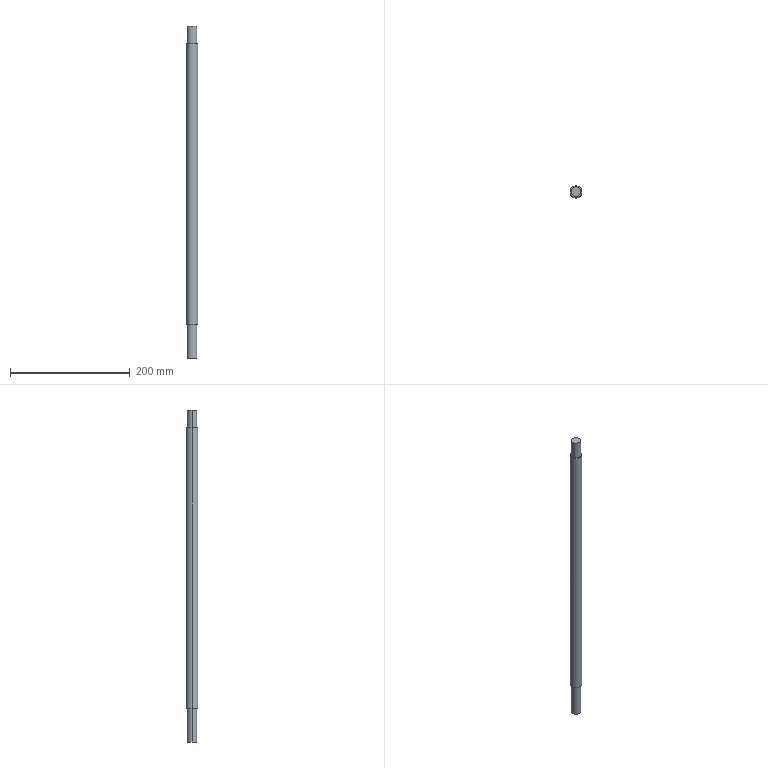Component | SolidWorks | LeadScrew-1 | 1 solid | 10 faces | box 20 x 20 x 555.57 mm | volume 164746 mm3 | cylinder 6 | plane 4 | commonest cylinder face diameters 16 x4 20 x2
build123d program:
from build123d import *

# Parameters (mm, degrees)
SKETCH1_R           = 10
BOSS_EXTRUDE1_DEPTH = 529
SKETCH2_R           = 10
SKETCH2_R_2         = 8
CUT_EXTRUDE1_DEPTH  = 30
CUT_EXTRUDE2_START  = -30
SKETCH3_R           = 10
SKETCH3_R_2         = 8
CUT_EXTRUDE2_DEPTH  = 30
MOVE_FACE1_BY       = 26.565


with BuildPart() as part:
    # Sketch1 → Boss-Extrude1 (new body)
    with BuildSketch(Plane.XY):
        with Locations((0, -208.707)):
            Circle(SKETCH1_R)
    extrude(amount=BOSS_EXTRUDE1_DEPTH)

    # Sketch2 → Cut-Extrude1 (cut)
    with BuildSketch(Plane(origin=(0, 0, 0), x_dir=(-1, 0, 0), z_dir=(0, 0, -1))):
        with Locations((0, -208.707)):
            Circle(SKETCH2_R)
        with Locations((0, -208.707)):
            Circle(SKETCH2_R_2, mode=Mode.SUBTRACT)
    extrude(amount=-CUT_EXTRUDE1_DEPTH, mode=Mode.SUBTRACT)

    # Sketch3 → Cut-Extrude2 (cut)
    with BuildSketch(Plane.XY.offset(529).offset(CUT_EXTRUDE2_START)):
        with Locations(Location((0, -208.707, 0), (0, 0, 180))):
            Circle(SKETCH3_R)
        with Locations(Location((0, -208.707, 0), (0, 0, 180))):
            Circle(SKETCH3_R_2, mode=Mode.SUBTRACT)
    extrude(amount=CUT_EXTRUDE2_DEPTH, mode=Mode.SUBTRACT)

    # Move Face1: a face moved outward by 26.565
    extrude(part.faces().sort_by_distance((0, -208.707, 529))[0], amount=MOVE_FACE1_BY, dir=(0, 0, 1))


solid = part.part

# Placed as in the assembly
solid = solid.moved(Location((0, -417.415, -102), (180, 0, 0)))
STEP:
#1=COLOUR_RGB('',0.7922,0.8196,0.9333);
#2=FILL_AREA_STYLE_COLOUR('',#1);
#3=FILL_AREA_STYLE('',(#2));
#4=SURFACE_STYLE_FILL_AREA(#3);
#5=SURFACE_SIDE_STYLE('',(#4));
#6=SURFACE_STYLE_USAGE(.BOTH.,#5);
#7=PRESENTATION_STYLE_ASSIGNMENT((#6));
#8=CARTESIAN_POINT('',(-0.315,-8.217,-23.661));
#9=VERTEX_POINT('',#8);
#10=CARTESIAN_POINT('',(0.315,-8.217,-23.661));
#11=VERTEX_POINT('',#10);
#12=CARTESIAN_POINT('',(0.,-8.217,-23.661));
#13=DIRECTION('',(0.,0.,-1.));
#14=DIRECTION('',(-1.,0.,0.));
#15=AXIS2_PLACEMENT_3D('',#12,#13,#14);
#16=CIRCLE('',#15,0.315);
#17=EDGE_CURVE('',#9,#11,#16,.T.);
#18=ORIENTED_EDGE('',*,*,#17,.T.);
#19=CARTESIAN_POINT('',(0.315,-8.217,-25.888));
#20=VERTEX_POINT('',#19);
#21=CARTESIAN_POINT('',(0.315,-8.217,-23.661));
#22=DIRECTION('',(0.,0.,-1.));
#23=VECTOR('',#22,39.37);
#24=LINE('',#21,#23);
#25=EDGE_CURVE('',#11,#20,#24,.T.);
#26=ORIENTED_EDGE('',*,*,#25,.T.);
#27=CARTESIAN_POINT('',(-0.315,-8.217,-25.888));
#28=VERTEX_POINT('',#27);
#29=CARTESIAN_POINT('',(0.,-8.217,-25.888));
#30=DIRECTION('',(0.,0.,-1.));
#31=DIRECTION('',(-1.,0.,0.));
#32=AXIS2_PLACEMENT_3D('',#29,#30,#31);
#33=CIRCLE('',#32,0.315);
#34=EDGE_CURVE('',#28,#20,#33,.T.);
#35=ORIENTED_EDGE('',*,*,#34,.F.);
#36=CARTESIAN_POINT('',(-0.315,-8.217,-23.661));
#37=DIRECTION('',(0.,0.,-1.));
#38=VECTOR('',#37,39.37);
#39=LINE('',#36,#38);
#40=EDGE_CURVE('',#9,#28,#39,.T.);
#41=ORIENTED_EDGE('',*,*,#40,.F.);
#42=EDGE_LOOP('',(#18,#26,#35,#41));
#43=FACE_OUTER_BOUND('',#42,.T.);
#44=CARTESIAN_POINT('',(0.,-8.217,-23.661));
#45=DIRECTION('',(0.,0.,-1.));
#46=DIRECTION('',(-1.,0.,0.));
#47=AXIS2_PLACEMENT_3D('',#44,#45,#46);
#48=CYLINDRICAL_SURFACE('',#47,0.315);
#49=ADVANCED_FACE('',(#43),#48,.T.);
#50=CARTESIAN_POINT('',(0.315,-8.217,-5.197));
#51=VERTEX_POINT('',#50);
#52=CARTESIAN_POINT('',(-0.315,-8.217,-5.197));
#53=VERTEX_POINT('',#52);
#54=CARTESIAN_POINT('',(0.,-8.217,-5.197));
#55=DIRECTION('',(0.,0.,1.));
#56=DIRECTION('',(1.,0.,0.));
#57=AXIS2_PLACEMENT_3D('',#54,#55,#56);
#58=CIRCLE('',#57,0.315);
#59=EDGE_CURVE('',#51,#53,#58,.T.);
#60=ORIENTED_EDGE('',*,*,#59,.T.);
#61=CARTESIAN_POINT('',(-0.315,-8.217,-4.016));
#62=VERTEX_POINT('',#61);
#63=CARTESIAN_POINT('',(-0.315,-8.217,-5.197));
#64=DIRECTION('',(0.,0.,1.));
#65=VECTOR('',#64,39.37);
#66=LINE('',#63,#65);
#67=EDGE_CURVE('',#53,#62,#66,.T.);
#68=ORIENTED_EDGE('',*,*,#67,.T.);
#69=CARTESIAN_POINT('',(0.315,-8.217,-4.016));
#70=VERTEX_POINT('',#69);
#71=CARTESIAN_POINT('',(0.,-8.217,-4.016));
#72=DIRECTION('',(0.,0.,1.));
#73=DIRECTION('',(1.,0.,0.));
#74=AXIS2_PLACEMENT_3D('',#71,#72,#73);
#75=CIRCLE('',#74,0.315);
#76=EDGE_CURVE('',#70,#62,#75,.T.);
#77=ORIENTED_EDGE('',*,*,#76,.F.);
#78=CARTESIAN_POINT('',(0.315,-8.217,-5.197));
#79=DIRECTION('',(0.,0.,1.));
#80=VECTOR('',#79,39.37);
#81=LINE('',#78,#80);
#82=EDGE_CURVE('',#51,#70,#81,.T.);
#83=ORIENTED_EDGE('',*,*,#82,.F.);
#84=EDGE_LOOP('',(#60,#68,#77,#83));
#85=FACE_OUTER_BOUND('',#84,.T.);
#86=CARTESIAN_POINT('',(0.,-8.217,-5.197));
#87=DIRECTION('',(0.,0.,1.));
#88=DIRECTION('',(1.,0.,0.));
#89=AXIS2_PLACEMENT_3D('',#86,#87,#88);
#90=CYLINDRICAL_SURFACE('',#89,0.315);
#91=ADVANCED_FACE('',(#85),#90,.T.);
#92=CARTESIAN_POINT('',(-0.3937,-8.217,-23.661));
#93=VERTEX_POINT('',#92);
#94=CARTESIAN_POINT('',(0.3937,-8.217,-23.661));
#95=VERTEX_POINT('',#94);
#96=CARTESIAN_POINT('',(0.,-8.217,-23.661));
#97=DIRECTION('',(0.,0.,-1.));
#98=DIRECTION('',(-1.,0.,0.));
#99=AXIS2_PLACEMENT_3D('',#96,#97,#98);
#100=CIRCLE('',#99,0.3937);
#101=EDGE_CURVE('',#93,#95,#100,.T.);
#102=ORIENTED_EDGE('',*,*,#101,.F.);
#103=CARTESIAN_POINT('',(-0.3937,-8.217,-5.197));
#104=VERTEX_POINT('',#103);
#105=CARTESIAN_POINT('',(-0.3937,-8.217,-24.843));
#106=DIRECTION('',(0.,0.,1.));
#107=VECTOR('',#106,39.37);
#108=LINE('',#105,#107);
#109=EDGE_CURVE('',#93,#104,#108,.T.);
#110=ORIENTED_EDGE('',*,*,#109,.T.);
#111=CARTESIAN_POINT('',(0.3937,-8.217,-5.197));
#112=VERTEX_POINT('',#111);
#113=CARTESIAN_POINT('',(0.,-8.217,-5.197));
#114=DIRECTION('',(0.,0.,1.));
#115=DIRECTION('',(1.,0.,0.));
#116=AXIS2_PLACEMENT_3D('',#113,#114,#115);
#117=CIRCLE('',#116,0.3937);
#118=EDGE_CURVE('',#112,#104,#117,.T.);
#119=ORIENTED_EDGE('',*,*,#118,.F.);
#120=CARTESIAN_POINT('',(0.3937,-8.217,-24.843));
#121=DIRECTION('',(0.,0.,1.));
#122=VECTOR('',#121,39.37);
#123=LINE('',#120,#122);
#124=EDGE_CURVE('',#95,#112,#123,.T.);
#125=ORIENTED_EDGE('',*,*,#124,.F.);
#126=EDGE_LOOP('',(#102,#110,#119,#125));
#127=FACE_OUTER_BOUND('',#126,.T.);
#128=CARTESIAN_POINT('',(0.,-8.217,-24.843));
#129=DIRECTION('',(0.,0.,1.));
#130=DIRECTION('',(1.,0.,0.));
#131=AXIS2_PLACEMENT_3D('',#128,#129,#130);
#132=CYLINDRICAL_SURFACE('',#131,0.3937);
#133=ADVANCED_FACE('',(#127),#132,.T.);
#134=ORIENTED_EDGE('',*,*,#109,.F.);
#135=CARTESIAN_POINT('',(0.,-8.217,-23.661));
#136=DIRECTION('',(0.,0.,-1.));
#137=DIRECTION('',(-1.,0.,0.));
#138=AXIS2_PLACEMENT_3D('',#135,#136,#137);
#139=CIRCLE('',#138,0.3937);
#140=EDGE_CURVE('',#95,#93,#139,.T.);
#141=ORIENTED_EDGE('',*,*,#140,.F.);
#142=ORIENTED_EDGE('',*,*,#124,.T.);
#143=CARTESIAN_POINT('',(0.,-8.217,-5.197));
#144=DIRECTION('',(0.,0.,1.));
#145=DIRECTION('',(1.,0.,0.));
#146=AXIS2_PLACEMENT_3D('',#143,#144,#145);
#147=CIRCLE('',#146,0.3937);
#148=EDGE_CURVE('',#104,#112,#147,.T.);
#149=ORIENTED_EDGE('',*,*,#148,.F.);
#150=EDGE_LOOP('',(#134,#141,#142,#149));
#151=FACE_OUTER_BOUND('',#150,.T.);
#152=CARTESIAN_POINT('',(0.,-8.217,-24.843));
#153=DIRECTION('',(0.,0.,1.));
#154=DIRECTION('',(1.,0.,0.));
#155=AXIS2_PLACEMENT_3D('',#152,#153,#154);
#156=CYLINDRICAL_SURFACE('',#155,0.3937);
#157=ADVANCED_FACE('',(#151),#156,.T.);
#158=ORIENTED_EDGE('',*,*,#59,.F.);
#159=CARTESIAN_POINT('',(0.,-8.217,-5.197));
#160=DIRECTION('',(0.,0.,1.));
#161=DIRECTION('',(1.,0.,0.));
#162=AXIS2_PLACEMENT_3D('',#159,#160,#161);
#163=CIRCLE('',#162,0.315);
#164=EDGE_CURVE('',#53,#51,#163,.T.);
#165=ORIENTED_EDGE('',*,*,#164,.F.);
#166=EDGE_LOOP('',(#158,#165));
#167=FACE_BOUND('',#166,.T.);
#168=ORIENTED_EDGE('',*,*,#118,.T.);
#169=ORIENTED_EDGE('',*,*,#148,.T.);
#170=EDGE_LOOP('',(#168,#169));
#171=FACE_OUTER_BOUND('',#170,.T.);
#172=CARTESIAN_POINT('',(0.,-8.217,-5.197));
#173=DIRECTION('',(0.,0.,1.));
#174=DIRECTION('',(1.,0.,0.));
#175=AXIS2_PLACEMENT_3D('',#172,#173,#174);
#176=PLANE('',#175);
#177=ADVANCED_FACE('',(#167,#171),#176,.T.);
#178=ORIENTED_EDGE('',*,*,#67,.F.);
#179=ORIENTED_EDGE('',*,*,#164,.T.);
#180=ORIENTED_EDGE('',*,*,#82,.T.);
#181=CARTESIAN_POINT('',(0.,-8.217,-4.016));
#182=DIRECTION('',(0.,0.,1.));
#183=DIRECTION('',(1.,0.,0.));
#184=AXIS2_PLACEMENT_3D('',#181,#182,#183);
#185=CIRCLE('',#184,0.315);
#186=EDGE_CURVE('',#62,#70,#185,.T.);
#187=ORIENTED_EDGE('',*,*,#186,.F.);
#188=EDGE_LOOP('',(#178,#179,#180,#187));
#189=FACE_OUTER_BOUND('',#188,.T.);
#190=CARTESIAN_POINT('',(0.,-8.217,-5.197));
#191=DIRECTION('',(0.,0.,1.));
#192=DIRECTION('',(1.,0.,0.));
#193=AXIS2_PLACEMENT_3D('',#190,#191,#192);
#194=CYLINDRICAL_SURFACE('',#193,0.315);
#195=ADVANCED_FACE('',(#189),#194,.T.);
#196=ORIENTED_EDGE('',*,*,#76,.T.);
#197=ORIENTED_EDGE('',*,*,#186,.T.);
#198=EDGE_LOOP('',(#196,#197));
#199=FACE_OUTER_BOUND('',#198,.T.);
#200=CARTESIAN_POINT('',(0.,-8.217,-4.016));
#201=DIRECTION('',(0.,0.,-1.));
#202=DIRECTION('',(-1.,0.,0.));
#203=AXIS2_PLACEMENT_3D('',#200,#201,#202);
#204=PLANE('',#203);
#205=ADVANCED_FACE('',(#199),#204,.F.);
#206=ORIENTED_EDGE('',*,*,#25,.F.);
#207=CARTESIAN_POINT('',(0.,-8.217,-23.661));
#208=DIRECTION('',(0.,0.,-1.));
#209=DIRECTION('',(-1.,0.,0.));
#210=AXIS2_PLACEMENT_3D('',#207,#208,#209);
#211=CIRCLE('',#210,0.315);
#212=EDGE_CURVE('',#11,#9,#211,.T.);
#213=ORIENTED_EDGE('',*,*,#212,.T.);
#214=ORIENTED_EDGE('',*,*,#40,.T.);
#215=CARTESIAN_POINT('',(0.,-8.217,-25.888));
#216=DIRECTION('',(0.,0.,-1.));
#217=DIRECTION('',(-1.,0.,0.));
#218=AXIS2_PLACEMENT_3D('',#215,#216,#217);
#219=CIRCLE('',#218,0.315);
#220=EDGE_CURVE('',#20,#28,#219,.T.);
#221=ORIENTED_EDGE('',*,*,#220,.F.);
#222=EDGE_LOOP('',(#206,#213,#214,#221));
#223=FACE_OUTER_BOUND('',#222,.T.);
#224=CARTESIAN_POINT('',(0.,-8.217,-23.661));
#225=DIRECTION('',(0.,0.,-1.));
#226=DIRECTION('',(-1.,0.,0.));
#227=AXIS2_PLACEMENT_3D('',#224,#225,#226);
#228=CYLINDRICAL_SURFACE('',#227,0.315);
#229=ADVANCED_FACE('',(#223),#228,.T.);
#230=ORIENTED_EDGE('',*,*,#17,.F.);
#231=ORIENTED_EDGE('',*,*,#212,.F.);
#232=EDGE_LOOP('',(#230,#231));
#233=FACE_BOUND('',#232,.T.);
#234=ORIENTED_EDGE('',*,*,#140,.T.);
#235=ORIENTED_EDGE('',*,*,#101,.T.);
#236=EDGE_LOOP('',(#234,#235));
#237=FACE_OUTER_BOUND('',#236,.T.);
#238=CARTESIAN_POINT('',(0.,0.,-23.661));
#239=DIRECTION('',(0.,0.,-1.));
#240=DIRECTION('',(-1.,0.,0.));
#241=AXIS2_PLACEMENT_3D('',#238,#239,#240);
#242=PLANE('',#241);
#243=ADVANCED_FACE('',(#233,#237),#242,.T.);
#244=ORIENTED_EDGE('',*,*,#34,.T.);
#245=ORIENTED_EDGE('',*,*,#220,.T.);
#246=EDGE_LOOP('',(#244,#245));
#247=FACE_OUTER_BOUND('',#246,.T.);
#248=CARTESIAN_POINT('',(0.,-8.217,-25.888));
#249=DIRECTION('',(0.,0.,-1.));
#250=DIRECTION('',(-1.,0.,0.));
#251=AXIS2_PLACEMENT_3D('',#248,#249,#250);
#252=PLANE('',#251);
#253=ADVANCED_FACE('',(#247),#252,.T.);
#254=CLOSED_SHELL('',(#49,#91,#133,#157,#177,#195,#205,#229,#243,#253));
#255=MANIFOLD_SOLID_BREP('',#254);
#256=STYLED_ITEM('',(#7),#255);
#257=(LENGTH_UNIT()NAMED_UNIT(*)SI_UNIT($,.METRE.));
#258=LENGTH_MEASURE_WITH_UNIT(LENGTH_MEASURE(0.0254),#257);
#259=DIMENSIONAL_EXPONENTS(1.,0.,0.,0.,0.,0.,0.);
#260=(CONVERSION_BASED_UNIT('',#258)LENGTH_UNIT()NAMED_UNIT(#259));
#261=UNCERTAINTY_MEASURE_WITH_UNIT(LENGTH_MEASURE(0.00001),#260,'','');
#262=(NAMED_UNIT(*)PLANE_ANGLE_UNIT()SI_UNIT($,.RADIAN.));
#263=(NAMED_UNIT(*)SI_UNIT($,.STERADIAN.)SOLID_ANGLE_UNIT());
#264=(GEOMETRIC_REPRESENTATION_CONTEXT(3)GLOBAL_UNCERTAINTY_ASSIGNED_CONTEXT((#261))GLOBAL_UNIT_ASSIGNED_CONTEXT((#260,#262,#263))REPRESENTATION_CONTEXT('',''));
#265=MECHANICAL_DESIGN_GEOMETRIC_PRESENTATION_REPRESENTATION('',(#256),#264);
#266=PRESENTATION_LAYER_ASSIGNMENT('','',(#256));
#267=CARTESIAN_POINT('',(0.,0.,0.));
#268=DIRECTION('',(0.,0.,1.));
#269=DIRECTION('',(1.,0.,0.));
#270=AXIS2_PLACEMENT_3D('',#267,#268,#269);
#271=(LENGTH_UNIT()NAMED_UNIT(*)SI_UNIT($,.METRE.));
#272=LENGTH_MEASURE_WITH_UNIT(LENGTH_MEASURE(0.0254),#271);
#273=DIMENSIONAL_EXPONENTS(1.,0.,0.,0.,0.,0.,0.);
#274=(CONVERSION_BASED_UNIT('',#272)LENGTH_UNIT()NAMED_UNIT(#273));
#275=UNCERTAINTY_MEASURE_WITH_UNIT(LENGTH_MEASURE(0.00001),#274,'','');
#276=(NAMED_UNIT(*)PLANE_ANGLE_UNIT()SI_UNIT($,.RADIAN.));
#277=(NAMED_UNIT(*)SI_UNIT($,.STERADIAN.)SOLID_ANGLE_UNIT());
#278=(GEOMETRIC_REPRESENTATION_CONTEXT(3)GLOBAL_UNCERTAINTY_ASSIGNED_CONTEXT((#275))GLOBAL_UNIT_ASSIGNED_CONTEXT((#274,#276,#277))REPRESENTATION_CONTEXT('',''));
#279=ADVANCED_BREP_SHAPE_REPRESENTATION('',(#255,#270),#278);